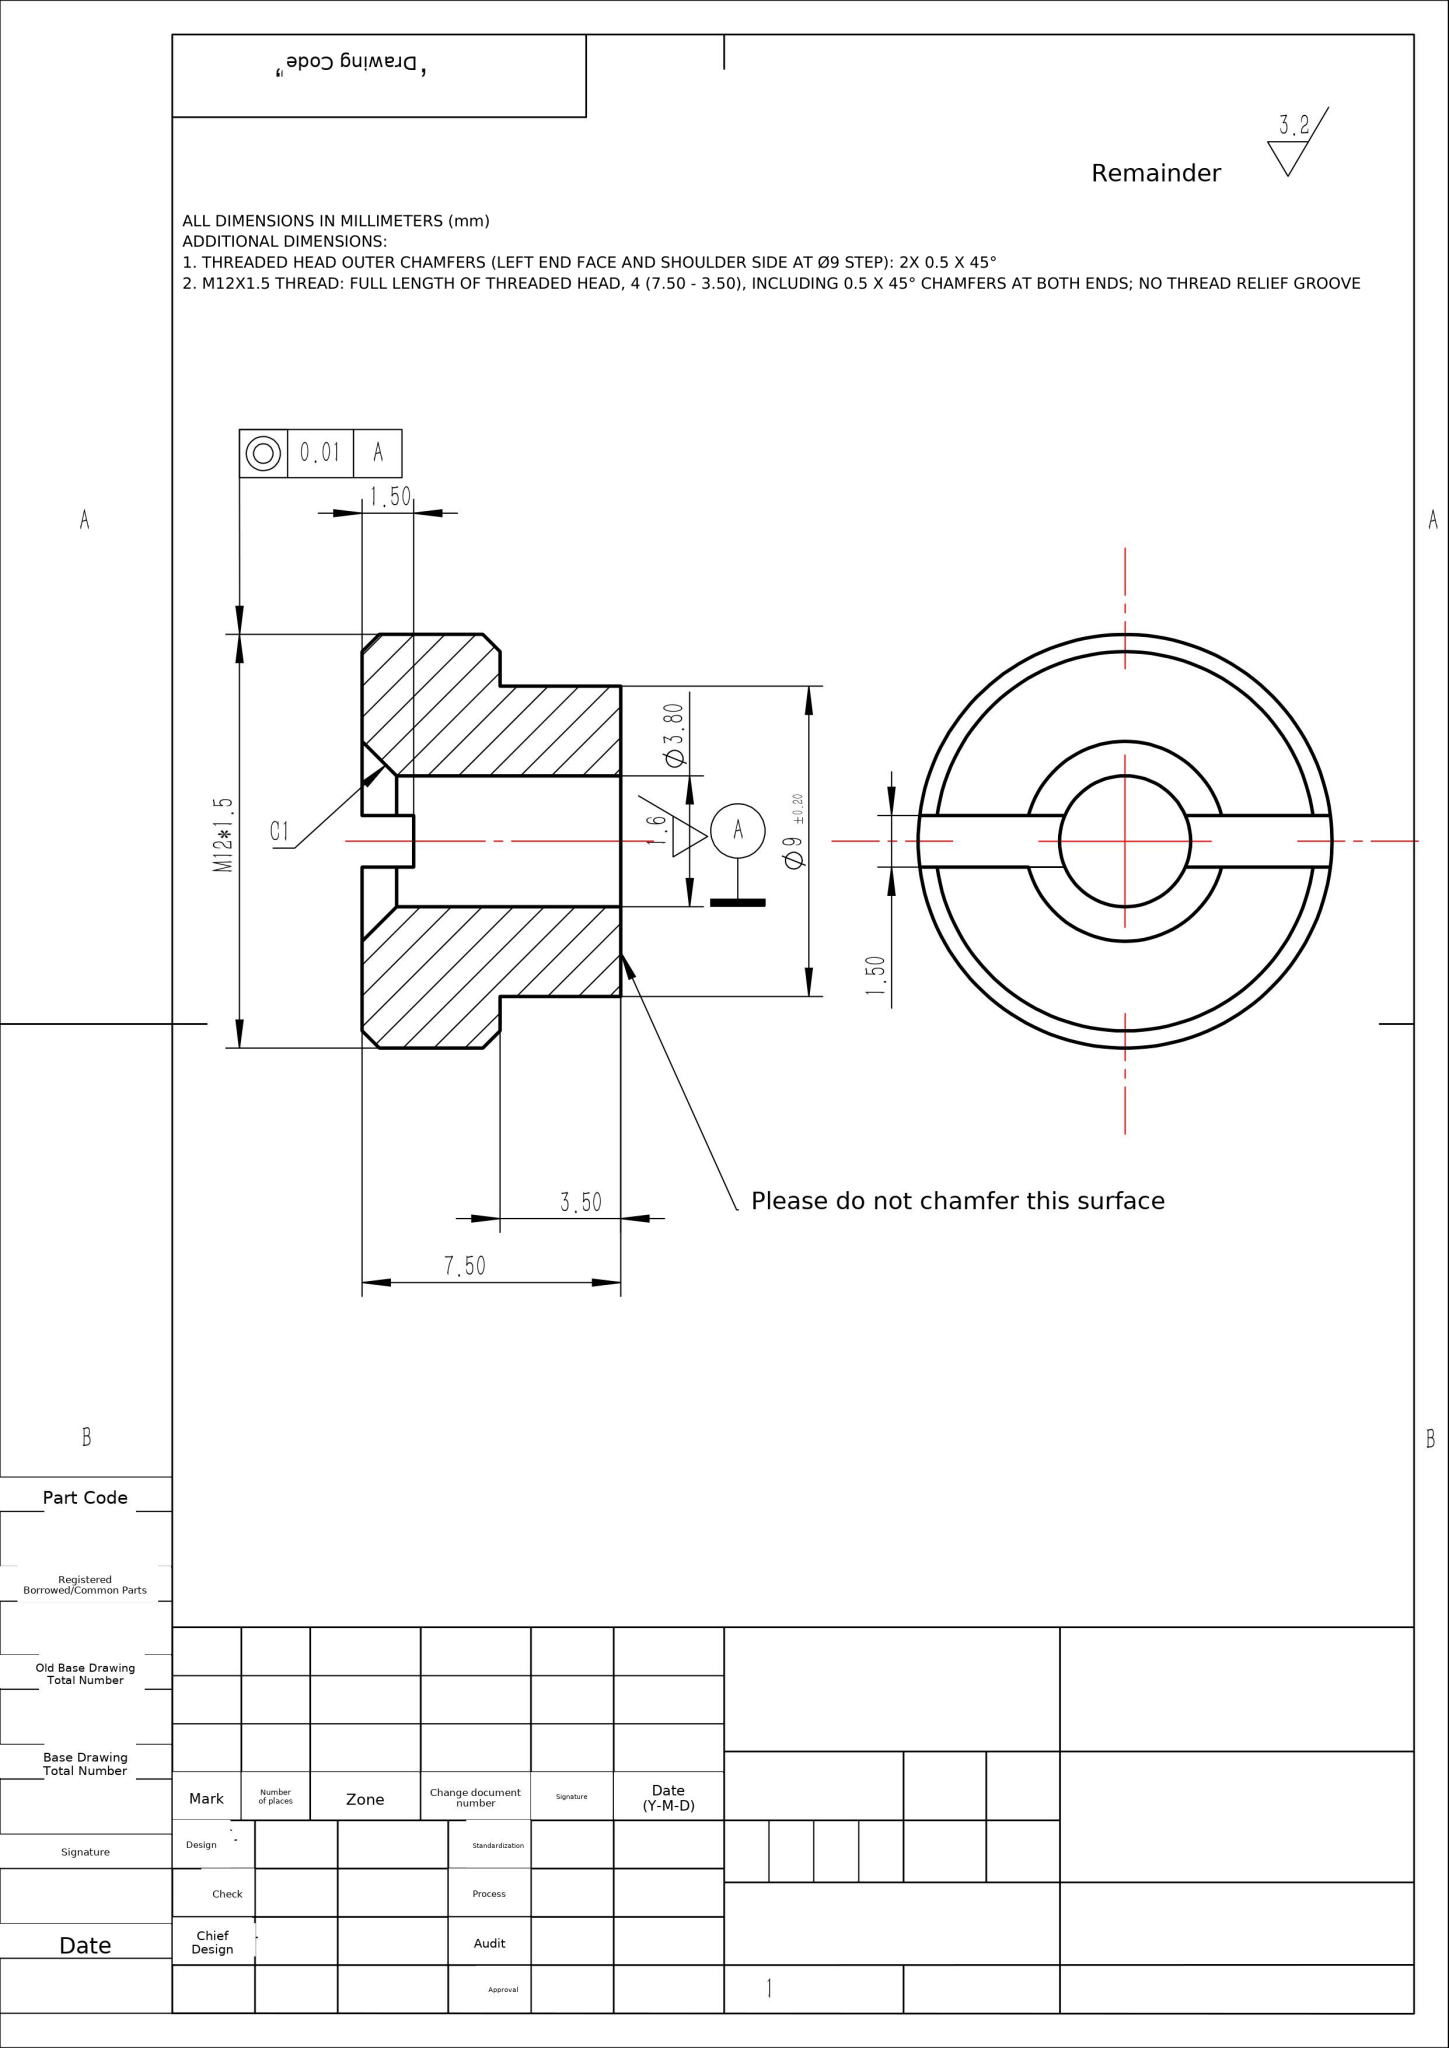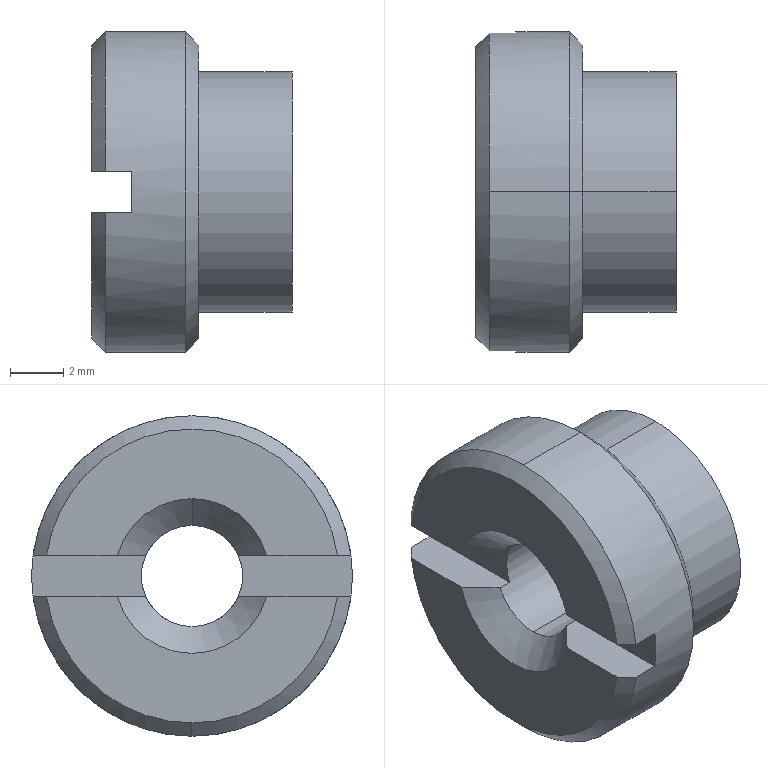Part | NX | mm | 1 solid | 24 faces | box 7.5 x 12 x 12 mm | volume 557 mm3 | plane 10 | cone 8 | cylinder 6 | commonest cylinder face diameters 3.8 x2 9 x2 12 x2
STEP:
#1=COLOUR_RGB('',0.6471,0.5176,0.);
#2=FILL_AREA_STYLE_COLOUR('',#1);
#3=FILL_AREA_STYLE('',(#2));
#4=SURFACE_STYLE_FILL_AREA(#3);
#5=SURFACE_SIDE_STYLE('',(#4));
#6=SURFACE_STYLE_USAGE(.BOTH.,#5);
#7=PRESENTATION_STYLE_ASSIGNMENT((#6));
#8=CARTESIAN_POINT('',(1.,-1.746,0.75));
#9=VERTEX_POINT('',#8);
#10=CARTESIAN_POINT('',(1.,-0.,1.9));
#11=VERTEX_POINT('',#10);
#12=CARTESIAN_POINT('',(1.,0.,0.));
#13=DIRECTION('',(-1.,0.,0.));
#14=DIRECTION('',(0.,0.,-1.));
#15=AXIS2_PLACEMENT_3D('',#12,#13,#14);
#16=CIRCLE('',#15,1.9);
#17=EDGE_CURVE('',#9,#11,#16,.T.);
#18=ORIENTED_EDGE('',*,*,#17,.T.);
#19=CARTESIAN_POINT('',(7.5,0.,1.9));
#20=VERTEX_POINT('',#19);
#21=CARTESIAN_POINT('',(0.,0.,1.9));
#22=DIRECTION('',(1.,0.,0.));
#23=VECTOR('',#22,1000.);
#24=LINE('',#21,#23);
#25=EDGE_CURVE('',#11,#20,#24,.T.);
#26=ORIENTED_EDGE('',*,*,#25,.T.);
#27=CARTESIAN_POINT('',(7.5,0.,-1.9));
#28=VERTEX_POINT('',#27);
#29=CARTESIAN_POINT('',(7.5,0.,0.));
#30=DIRECTION('',(1.,0.,0.));
#31=DIRECTION('',(0.,0.,-1.));
#32=AXIS2_PLACEMENT_3D('',#29,#30,#31);
#33=CIRCLE('',#32,1.9);
#34=EDGE_CURVE('',#20,#28,#33,.T.);
#35=ORIENTED_EDGE('',*,*,#34,.T.);
#36=CARTESIAN_POINT('',(1.,0.,-1.9));
#37=VERTEX_POINT('',#36);
#38=CARTESIAN_POINT('',(0.,0.,-1.9));
#39=DIRECTION('',(1.,0.,0.));
#40=VECTOR('',#39,1000.);
#41=LINE('',#38,#40);
#42=EDGE_CURVE('',#37,#28,#41,.T.);
#43=ORIENTED_EDGE('',*,*,#42,.F.);
#44=CARTESIAN_POINT('',(1.,-1.746,-0.75));
#45=VERTEX_POINT('',#44);
#46=CARTESIAN_POINT('',(1.,0.,0.));
#47=DIRECTION('',(-1.,0.,0.));
#48=DIRECTION('',(0.,0.,-1.));
#49=AXIS2_PLACEMENT_3D('',#46,#47,#48);
#50=CIRCLE('',#49,1.9);
#51=EDGE_CURVE('',#37,#45,#50,.T.);
#52=ORIENTED_EDGE('',*,*,#51,.T.);
#53=CARTESIAN_POINT('',(1.5,-1.746,-0.75));
#54=VERTEX_POINT('',#53);
#55=CARTESIAN_POINT('',(0.,-1.746,-0.75));
#56=DIRECTION('',(1.,0.,0.));
#57=VECTOR('',#56,1000.);
#58=LINE('',#55,#57);
#59=EDGE_CURVE('',#45,#54,#58,.T.);
#60=ORIENTED_EDGE('',*,*,#59,.T.);
#61=CARTESIAN_POINT('',(1.5,-1.746,0.75));
#62=VERTEX_POINT('',#61);
#63=CARTESIAN_POINT('',(1.5,0.,0.));
#64=DIRECTION('',(-1.,0.,0.));
#65=DIRECTION('',(0.,0.,-1.));
#66=AXIS2_PLACEMENT_3D('',#63,#64,#65);
#67=CIRCLE('',#66,1.9);
#68=EDGE_CURVE('',#54,#62,#67,.T.);
#69=ORIENTED_EDGE('',*,*,#68,.T.);
#70=CARTESIAN_POINT('',(0.,-1.746,0.75));
#71=DIRECTION('',(-1.,0.,0.));
#72=VECTOR('',#71,1000.);
#73=LINE('',#70,#72);
#74=EDGE_CURVE('',#62,#9,#73,.T.);
#75=ORIENTED_EDGE('',*,*,#74,.T.);
#76=EDGE_LOOP('',(#18,#26,#35,#43,#52,#60,#69,#75));
#77=FACE_OUTER_BOUND('',#76,.T.);
#78=CARTESIAN_POINT('',(0.,0.,0.));
#79=DIRECTION('',(1.,0.,0.));
#80=DIRECTION('',(0.,0.,-1.));
#81=AXIS2_PLACEMENT_3D('',#78,#79,#80);
#82=CYLINDRICAL_SURFACE('',#81,1.9);
#83=ADVANCED_FACE('',(#77),#82,.F.);
#84=CARTESIAN_POINT('',(4.,0.,-5.5));
#85=VERTEX_POINT('',#84);
#86=CARTESIAN_POINT('',(4.,-0.,5.5));
#87=VERTEX_POINT('',#86);
#88=CARTESIAN_POINT('',(4.,0.,0.));
#89=DIRECTION('',(1.,0.,0.));
#90=DIRECTION('',(0.,0.,-1.));
#91=AXIS2_PLACEMENT_3D('',#88,#89,#90);
#92=CIRCLE('',#91,5.5);
#93=EDGE_CURVE('',#85,#87,#92,.T.);
#94=ORIENTED_EDGE('',*,*,#93,.F.);
#95=CARTESIAN_POINT('',(3.5,0.,-6.));
#96=VERTEX_POINT('',#95);
#97=CARTESIAN_POINT('',(4.,0.,-5.5));
#98=DIRECTION('',(-0.7071,0.,-0.7071));
#99=VECTOR('',#98,1000.);
#100=LINE('',#97,#99);
#101=EDGE_CURVE('',#85,#96,#100,.T.);
#102=ORIENTED_EDGE('',*,*,#101,.T.);
#103=CARTESIAN_POINT('',(3.5,-0.,6.));
#104=VERTEX_POINT('',#103);
#105=CARTESIAN_POINT('',(3.5,0.,0.));
#106=DIRECTION('',(-1.,0.,0.));
#107=DIRECTION('',(0.,0.,-1.));
#108=AXIS2_PLACEMENT_3D('',#105,#106,#107);
#109=CIRCLE('',#108,6.);
#110=EDGE_CURVE('',#104,#96,#109,.T.);
#111=ORIENTED_EDGE('',*,*,#110,.F.);
#112=CARTESIAN_POINT('',(4.,-0.,5.5));
#113=DIRECTION('',(-0.7071,-0.,0.7071));
#114=VECTOR('',#113,1000.);
#115=LINE('',#112,#114);
#116=EDGE_CURVE('',#87,#104,#115,.T.);
#117=ORIENTED_EDGE('',*,*,#116,.F.);
#118=EDGE_LOOP('',(#94,#102,#111,#117));
#119=FACE_OUTER_BOUND('',#118,.T.);
#120=CARTESIAN_POINT('',(4.,0.,0.));
#121=DIRECTION('',(-1.,0.,0.));
#122=DIRECTION('',(0.,-0.,1.));
#123=AXIS2_PLACEMENT_3D('',#120,#121,#122);
#124=CONICAL_SURFACE('',#123,5.5,0.7854);
#125=ADVANCED_FACE('',(#119),#124,.T.);
#126=CARTESIAN_POINT('',(0.,0.,-5.5));
#127=VERTEX_POINT('',#126);
#128=CARTESIAN_POINT('',(0.,-5.449,-0.75));
#129=VERTEX_POINT('',#128);
#130=CARTESIAN_POINT('',(0.,0.,0.));
#131=DIRECTION('',(-1.,0.,0.));
#132=DIRECTION('',(0.,0.,-1.));
#133=AXIS2_PLACEMENT_3D('',#130,#131,#132);
#134=CIRCLE('',#133,5.5);
#135=EDGE_CURVE('',#127,#129,#134,.T.);
#136=ORIENTED_EDGE('',*,*,#135,.F.);
#137=CARTESIAN_POINT('',(0.5,0.,-6.));
#138=VERTEX_POINT('',#137);
#139=CARTESIAN_POINT('',(0.5,0.,-6.));
#140=DIRECTION('',(0.7071,0.,-0.7071));
#141=VECTOR('',#140,1000.);
#142=LINE('',#139,#141);
#143=EDGE_CURVE('',#127,#138,#142,.T.);
#144=ORIENTED_EDGE('',*,*,#143,.T.);
#145=CARTESIAN_POINT('',(0.5,-5.953,-0.75));
#146=VERTEX_POINT('',#145);
#147=CARTESIAN_POINT('',(0.5,0.,0.));
#148=DIRECTION('',(1.,0.,0.));
#149=DIRECTION('',(0.,0.,-1.));
#150=AXIS2_PLACEMENT_3D('',#147,#148,#149);
#151=CIRCLE('',#150,6.);
#152=EDGE_CURVE('',#146,#138,#151,.T.);
#153=ORIENTED_EDGE('',*,*,#152,.F.);
#154=CARTESIAN_POINT('',(0.,-5.449,-0.75));
#155=CARTESIAN_POINT('',(0.1666,-5.617,-0.75));
#156=CARTESIAN_POINT('',(0.3333,-5.785,-0.75));
#157=CARTESIAN_POINT('',(0.5,-5.953,-0.75));
#158=B_SPLINE_CURVE_WITH_KNOTS('',3,(#154,#155,#156,#157),.UNSPECIFIED.,.F.,.F.,(4,4),(0.02551,0.02623),.UNSPECIFIED.);
#159=EDGE_CURVE('',#129,#146,#158,.T.);
#160=ORIENTED_EDGE('',*,*,#159,.F.);
#161=EDGE_LOOP('',(#136,#144,#153,#160));
#162=FACE_OUTER_BOUND('',#161,.T.);
#163=CARTESIAN_POINT('',(0.5,0.,0.));
#164=DIRECTION('',(1.,0.,0.));
#165=DIRECTION('',(0.,0.,-1.));
#166=AXIS2_PLACEMENT_3D('',#163,#164,#165);
#167=CONICAL_SURFACE('',#166,6.,0.7854);
#168=ADVANCED_FACE('',(#162),#167,.T.);
#169=CARTESIAN_POINT('',(7.5,0.,-4.5));
#170=VERTEX_POINT('',#169);
#171=CARTESIAN_POINT('',(7.5,-0.,4.5));
#172=VERTEX_POINT('',#171);
#173=CARTESIAN_POINT('',(7.5,0.,0.));
#174=DIRECTION('',(1.,0.,0.));
#175=DIRECTION('',(0.,0.,-1.));
#176=AXIS2_PLACEMENT_3D('',#173,#174,#175);
#177=CIRCLE('',#176,4.5);
#178=EDGE_CURVE('',#170,#172,#177,.T.);
#179=ORIENTED_EDGE('',*,*,#178,.F.);
#180=CARTESIAN_POINT('',(4.,0.,-4.5));
#181=VERTEX_POINT('',#180);
#182=CARTESIAN_POINT('',(7.5,0.,-4.5));
#183=DIRECTION('',(-1.,0.,0.));
#184=VECTOR('',#183,1000.);
#185=LINE('',#182,#184);
#186=EDGE_CURVE('',#170,#181,#185,.T.);
#187=ORIENTED_EDGE('',*,*,#186,.T.);
#188=CARTESIAN_POINT('',(4.,-0.,4.5));
#189=VERTEX_POINT('',#188);
#190=CARTESIAN_POINT('',(4.,0.,0.));
#191=DIRECTION('',(1.,0.,0.));
#192=DIRECTION('',(0.,0.,-1.));
#193=AXIS2_PLACEMENT_3D('',#190,#191,#192);
#194=CIRCLE('',#193,4.5);
#195=EDGE_CURVE('',#181,#189,#194,.T.);
#196=ORIENTED_EDGE('',*,*,#195,.T.);
#197=CARTESIAN_POINT('',(7.5,-0.,4.5));
#198=DIRECTION('',(-1.,0.,0.));
#199=VECTOR('',#198,1000.);
#200=LINE('',#197,#199);
#201=EDGE_CURVE('',#172,#189,#200,.T.);
#202=ORIENTED_EDGE('',*,*,#201,.F.);
#203=EDGE_LOOP('',(#179,#187,#196,#202));
#204=FACE_OUTER_BOUND('',#203,.T.);
#205=CARTESIAN_POINT('',(7.5,0.,0.));
#206=DIRECTION('',(-1.,0.,0.));
#207=DIRECTION('',(0.,-0.,1.));
#208=AXIS2_PLACEMENT_3D('',#205,#206,#207);
#209=CYLINDRICAL_SURFACE('',#208,4.5);
#210=ADVANCED_FACE('',(#204),#209,.T.);
#211=ORIENTED_EDGE('',*,*,#110,.T.);
#212=CARTESIAN_POINT('',(4.,0.,-6.));
#213=DIRECTION('',(-1.,0.,0.));
#214=VECTOR('',#213,1000.);
#215=LINE('',#212,#214);
#216=EDGE_CURVE('',#96,#138,#215,.T.);
#217=ORIENTED_EDGE('',*,*,#216,.T.);
#218=CARTESIAN_POINT('',(0.5,5.953,-0.75));
#219=VERTEX_POINT('',#218);
#220=CARTESIAN_POINT('',(0.5,0.,0.));
#221=DIRECTION('',(1.,0.,0.));
#222=DIRECTION('',(0.,0.,-1.));
#223=AXIS2_PLACEMENT_3D('',#220,#221,#222);
#224=CIRCLE('',#223,6.);
#225=EDGE_CURVE('',#138,#219,#224,.T.);
#226=ORIENTED_EDGE('',*,*,#225,.T.);
#227=CARTESIAN_POINT('',(1.5,5.953,-0.75));
#228=VERTEX_POINT('',#227);
#229=CARTESIAN_POINT('',(4.,5.953,-0.75));
#230=DIRECTION('',(1.,0.,0.));
#231=VECTOR('',#230,1000.);
#232=LINE('',#229,#231);
#233=EDGE_CURVE('',#219,#228,#232,.T.);
#234=ORIENTED_EDGE('',*,*,#233,.T.);
#235=CARTESIAN_POINT('',(1.5,5.953,0.75));
#236=VERTEX_POINT('',#235);
#237=CARTESIAN_POINT('',(1.5,0.,0.));
#238=DIRECTION('',(1.,0.,0.));
#239=DIRECTION('',(0.,0.,-1.));
#240=AXIS2_PLACEMENT_3D('',#237,#238,#239);
#241=CIRCLE('',#240,6.);
#242=EDGE_CURVE('',#228,#236,#241,.T.);
#243=ORIENTED_EDGE('',*,*,#242,.T.);
#244=CARTESIAN_POINT('',(0.5,5.953,0.75));
#245=VERTEX_POINT('',#244);
#246=CARTESIAN_POINT('',(4.,5.953,0.75));
#247=DIRECTION('',(-1.,0.,0.));
#248=VECTOR('',#247,1000.);
#249=LINE('',#246,#248);
#250=EDGE_CURVE('',#236,#245,#249,.T.);
#251=ORIENTED_EDGE('',*,*,#250,.T.);
#252=CARTESIAN_POINT('',(0.5,-0.,6.));
#253=VERTEX_POINT('',#252);
#254=CARTESIAN_POINT('',(0.5,0.,0.));
#255=DIRECTION('',(1.,0.,0.));
#256=DIRECTION('',(0.,0.,-1.));
#257=AXIS2_PLACEMENT_3D('',#254,#255,#256);
#258=CIRCLE('',#257,6.);
#259=EDGE_CURVE('',#245,#253,#258,.T.);
#260=ORIENTED_EDGE('',*,*,#259,.T.);
#261=CARTESIAN_POINT('',(4.,-0.,6.));
#262=DIRECTION('',(-1.,0.,0.));
#263=VECTOR('',#262,1000.);
#264=LINE('',#261,#263);
#265=EDGE_CURVE('',#104,#253,#264,.T.);
#266=ORIENTED_EDGE('',*,*,#265,.F.);
#267=EDGE_LOOP('',(#211,#217,#226,#234,#243,#251,#260,#266));
#268=FACE_OUTER_BOUND('',#267,.T.);
#269=CARTESIAN_POINT('',(4.,0.,0.));
#270=DIRECTION('',(-1.,0.,0.));
#271=DIRECTION('',(0.,-0.,1.));
#272=AXIS2_PLACEMENT_3D('',#269,#270,#271);
#273=CYLINDRICAL_SURFACE('',#272,6.);
#274=ADVANCED_FACE('',(#268),#273,.T.);
#275=CARTESIAN_POINT('',(1.,1.746,0.75));
#276=VERTEX_POINT('',#275);
#277=CARTESIAN_POINT('',(1.,0.,0.));
#278=DIRECTION('',(-1.,0.,0.));
#279=DIRECTION('',(0.,0.,-1.));
#280=AXIS2_PLACEMENT_3D('',#277,#278,#279);
#281=CIRCLE('',#280,1.9);
#282=EDGE_CURVE('',#11,#276,#281,.T.);
#283=ORIENTED_EDGE('',*,*,#282,.F.);
#284=CARTESIAN_POINT('',(0.,-0.,2.9));
#285=VERTEX_POINT('',#284);
#286=CARTESIAN_POINT('',(0.,-0.,2.9));
#287=DIRECTION('',(-0.7071,-0.,0.7071));
#288=VECTOR('',#287,1000.);
#289=LINE('',#286,#288);
#290=EDGE_CURVE('',#11,#285,#289,.T.);
#291=ORIENTED_EDGE('',*,*,#290,.T.);
#292=CARTESIAN_POINT('',(0.,2.801,0.75));
#293=VERTEX_POINT('',#292);
#294=CARTESIAN_POINT('',(0.,0.,0.));
#295=DIRECTION('',(1.,0.,0.));
#296=DIRECTION('',(0.,0.,-1.));
#297=AXIS2_PLACEMENT_3D('',#294,#295,#296);
#298=CIRCLE('',#297,2.9);
#299=EDGE_CURVE('',#293,#285,#298,.T.);
#300=ORIENTED_EDGE('',*,*,#299,.F.);
#301=CARTESIAN_POINT('',(1.,1.746,0.75));
#302=CARTESIAN_POINT('',(0.6721,2.103,0.75));
#303=CARTESIAN_POINT('',(0.3368,2.453,0.75));
#304=CARTESIAN_POINT('',(0.,2.801,0.75));
#305=B_SPLINE_CURVE_WITH_KNOTS('',3,(#301,#302,#303,#304),.UNSPECIFIED.,.F.,.F.,(4,4),(0.0107,0.01214),.UNSPECIFIED.);
#306=EDGE_CURVE('',#276,#293,#305,.T.);
#307=ORIENTED_EDGE('',*,*,#306,.F.);
#308=EDGE_LOOP('',(#283,#291,#300,#307));
#309=FACE_OUTER_BOUND('',#308,.T.);
#310=CARTESIAN_POINT('',(0.,0.,0.));
#311=DIRECTION('',(-1.,0.,0.));
#312=DIRECTION('',(0.,-0.,1.));
#313=AXIS2_PLACEMENT_3D('',#310,#311,#312);
#314=CONICAL_SURFACE('',#313,2.9,0.7854);
#315=ADVANCED_FACE('',(#309),#314,.F.);
#316=CARTESIAN_POINT('',(0.,-5.449,0.75));
#317=VERTEX_POINT('',#316);
#318=CARTESIAN_POINT('',(0.,5.449,0.75));
#319=VERTEX_POINT('',#318);
#320=CARTESIAN_POINT('',(0.,0.,0.));
#321=DIRECTION('',(-1.,0.,0.));
#322=DIRECTION('',(0.,0.,-1.));
#323=AXIS2_PLACEMENT_3D('',#320,#321,#322);
#324=CIRCLE('',#323,5.5);
#325=EDGE_CURVE('',#317,#319,#324,.T.);
#326=ORIENTED_EDGE('',*,*,#325,.T.);
#327=CARTESIAN_POINT('',(0.,0.,0.75));
#328=DIRECTION('',(0.,-1.,-0.));
#329=VECTOR('',#328,1000.);
#330=LINE('',#327,#329);
#331=EDGE_CURVE('',#319,#293,#330,.T.);
#332=ORIENTED_EDGE('',*,*,#331,.T.);
#333=ORIENTED_EDGE('',*,*,#299,.T.);
#334=CARTESIAN_POINT('',(0.,-2.801,0.75));
#335=VERTEX_POINT('',#334);
#336=CARTESIAN_POINT('',(0.,0.,0.));
#337=DIRECTION('',(1.,0.,0.));
#338=DIRECTION('',(0.,0.,-1.));
#339=AXIS2_PLACEMENT_3D('',#336,#337,#338);
#340=CIRCLE('',#339,2.9);
#341=EDGE_CURVE('',#285,#335,#340,.T.);
#342=ORIENTED_EDGE('',*,*,#341,.T.);
#343=CARTESIAN_POINT('',(0.,0.,0.75));
#344=DIRECTION('',(0.,-1.,-0.));
#345=VECTOR('',#344,1000.);
#346=LINE('',#343,#345);
#347=EDGE_CURVE('',#335,#317,#346,.T.);
#348=ORIENTED_EDGE('',*,*,#347,.T.);
#349=EDGE_LOOP('',(#326,#332,#333,#342,#348));
#350=FACE_OUTER_BOUND('',#349,.T.);
#351=CARTESIAN_POINT('',(0.,0.,0.));
#352=DIRECTION('',(1.,0.,0.));
#353=DIRECTION('',(0.,0.,-1.));
#354=AXIS2_PLACEMENT_3D('',#351,#352,#353);
#355=PLANE('',#354);
#356=ADVANCED_FACE('',(#350),#355,.F.);
#357=CARTESIAN_POINT('',(0.5,-5.953,0.75));
#358=VERTEX_POINT('',#357);
#359=CARTESIAN_POINT('',(0.5,-5.953,0.75));
#360=CARTESIAN_POINT('',(0.3333,-5.785,0.75));
#361=CARTESIAN_POINT('',(0.1666,-5.617,0.75));
#362=CARTESIAN_POINT('',(0.,-5.449,0.75));
#363=B_SPLINE_CURVE_WITH_KNOTS('',3,(#359,#360,#361,#362),.UNSPECIFIED.,.F.,.F.,(4,4),(0.01021,0.01092),.UNSPECIFIED.);
#364=EDGE_CURVE('',#358,#317,#363,.T.);
#365=ORIENTED_EDGE('',*,*,#364,.F.);
#366=CARTESIAN_POINT('',(0.5,0.,0.));
#367=DIRECTION('',(1.,0.,0.));
#368=DIRECTION('',(0.,0.,-1.));
#369=AXIS2_PLACEMENT_3D('',#366,#367,#368);
#370=CIRCLE('',#369,6.);
#371=EDGE_CURVE('',#253,#358,#370,.T.);
#372=ORIENTED_EDGE('',*,*,#371,.F.);
#373=ORIENTED_EDGE('',*,*,#259,.F.);
#374=CARTESIAN_POINT('',(0.,5.449,0.75));
#375=CARTESIAN_POINT('',(0.1666,5.617,0.75));
#376=CARTESIAN_POINT('',(0.3333,5.785,0.75));
#377=CARTESIAN_POINT('',(0.5,5.953,0.75));
#378=B_SPLINE_CURVE_WITH_KNOTS('',3,(#374,#375,#376,#377),.UNSPECIFIED.,.F.,.F.,(4,4),(0.02551,0.02623),.UNSPECIFIED.);
#379=EDGE_CURVE('',#319,#245,#378,.T.);
#380=ORIENTED_EDGE('',*,*,#379,.F.);
#381=ORIENTED_EDGE('',*,*,#325,.F.);
#382=EDGE_LOOP('',(#365,#372,#373,#380,#381));
#383=FACE_OUTER_BOUND('',#382,.T.);
#384=CARTESIAN_POINT('',(0.5,0.,0.));
#385=DIRECTION('',(1.,0.,0.));
#386=DIRECTION('',(0.,0.,-1.));
#387=AXIS2_PLACEMENT_3D('',#384,#385,#386);
#388=CONICAL_SURFACE('',#387,6.,0.7854);
#389=ADVANCED_FACE('',(#383),#388,.T.);
#390=ORIENTED_EDGE('',*,*,#290,.F.);
#391=ORIENTED_EDGE('',*,*,#17,.F.);
#392=CARTESIAN_POINT('',(0.,-2.801,0.75));
#393=CARTESIAN_POINT('',(0.3367,-2.453,0.75));
#394=CARTESIAN_POINT('',(0.672,-2.103,0.75));
#395=CARTESIAN_POINT('',(1.,-1.746,0.75));
#396=B_SPLINE_CURVE_WITH_KNOTS('',3,(#392,#393,#394,#395),.UNSPECIFIED.,.F.,.F.,(4,4),(0.005033,0.006487),.UNSPECIFIED.);
#397=EDGE_CURVE('',#335,#9,#396,.T.);
#398=ORIENTED_EDGE('',*,*,#397,.F.);
#399=ORIENTED_EDGE('',*,*,#341,.F.);
#400=EDGE_LOOP('',(#390,#391,#398,#399));
#401=FACE_OUTER_BOUND('',#400,.T.);
#402=CARTESIAN_POINT('',(0.,0.,0.));
#403=DIRECTION('',(-1.,0.,0.));
#404=DIRECTION('',(0.,-0.,1.));
#405=AXIS2_PLACEMENT_3D('',#402,#403,#404);
#406=CONICAL_SURFACE('',#405,2.9,0.7854);
#407=ADVANCED_FACE('',(#401),#406,.F.);
#408=CARTESIAN_POINT('',(4.,0.,0.));
#409=DIRECTION('',(1.,0.,0.));
#410=DIRECTION('',(0.,0.,-1.));
#411=AXIS2_PLACEMENT_3D('',#408,#409,#410);
#412=CIRCLE('',#411,5.5);
#413=EDGE_CURVE('',#87,#85,#412,.T.);
#414=ORIENTED_EDGE('',*,*,#413,.T.);
#415=ORIENTED_EDGE('',*,*,#93,.T.);
#416=EDGE_LOOP('',(#414,#415));
#417=FACE_OUTER_BOUND('',#416,.T.);
#418=CARTESIAN_POINT('',(4.,0.,0.));
#419=DIRECTION('',(1.,0.,0.));
#420=DIRECTION('',(0.,0.,-1.));
#421=AXIS2_PLACEMENT_3D('',#418,#419,#420);
#422=CIRCLE('',#421,4.5);
#423=EDGE_CURVE('',#189,#181,#422,.T.);
#424=ORIENTED_EDGE('',*,*,#423,.F.);
#425=ORIENTED_EDGE('',*,*,#195,.F.);
#426=EDGE_LOOP('',(#424,#425));
#427=FACE_BOUND('',#426,.T.);
#428=CARTESIAN_POINT('',(4.,0.,0.));
#429=DIRECTION('',(1.,0.,0.));
#430=DIRECTION('',(0.,0.,-1.));
#431=AXIS2_PLACEMENT_3D('',#428,#429,#430);
#432=PLANE('',#431);
#433=ADVANCED_FACE('',(#417,#427),#432,.T.);
#434=ORIENTED_EDGE('',*,*,#216,.F.);
#435=CARTESIAN_POINT('',(3.5,0.,0.));
#436=DIRECTION('',(-1.,0.,0.));
#437=DIRECTION('',(0.,0.,-1.));
#438=AXIS2_PLACEMENT_3D('',#435,#436,#437);
#439=CIRCLE('',#438,6.);
#440=EDGE_CURVE('',#96,#104,#439,.T.);
#441=ORIENTED_EDGE('',*,*,#440,.T.);
#442=ORIENTED_EDGE('',*,*,#265,.T.);
#443=ORIENTED_EDGE('',*,*,#371,.T.);
#444=CARTESIAN_POINT('',(1.5,-5.953,0.75));
#445=VERTEX_POINT('',#444);
#446=CARTESIAN_POINT('',(4.,-5.953,0.75));
#447=DIRECTION('',(1.,0.,0.));
#448=VECTOR('',#447,1000.);
#449=LINE('',#446,#448);
#450=EDGE_CURVE('',#358,#445,#449,.T.);
#451=ORIENTED_EDGE('',*,*,#450,.T.);
#452=CARTESIAN_POINT('',(1.5,-5.953,-0.75));
#453=VERTEX_POINT('',#452);
#454=CARTESIAN_POINT('',(1.5,0.,0.));
#455=DIRECTION('',(1.,0.,0.));
#456=DIRECTION('',(0.,0.,-1.));
#457=AXIS2_PLACEMENT_3D('',#454,#455,#456);
#458=CIRCLE('',#457,6.);
#459=EDGE_CURVE('',#445,#453,#458,.T.);
#460=ORIENTED_EDGE('',*,*,#459,.T.);
#461=CARTESIAN_POINT('',(4.,-5.953,-0.75));
#462=DIRECTION('',(-1.,0.,0.));
#463=VECTOR('',#462,1000.);
#464=LINE('',#461,#463);
#465=EDGE_CURVE('',#453,#146,#464,.T.);
#466=ORIENTED_EDGE('',*,*,#465,.T.);
#467=ORIENTED_EDGE('',*,*,#152,.T.);
#468=EDGE_LOOP('',(#434,#441,#442,#443,#451,#460,#466,#467));
#469=FACE_OUTER_BOUND('',#468,.T.);
#470=CARTESIAN_POINT('',(4.,0.,0.));
#471=DIRECTION('',(-1.,0.,0.));
#472=DIRECTION('',(0.,-0.,1.));
#473=AXIS2_PLACEMENT_3D('',#470,#471,#472);
#474=CYLINDRICAL_SURFACE('',#473,6.);
#475=ADVANCED_FACE('',(#469),#474,.T.);
#476=CARTESIAN_POINT('',(0.,5.449,-0.75));
#477=VERTEX_POINT('',#476);
#478=CARTESIAN_POINT('',(0.,0.,0.));
#479=DIRECTION('',(-1.,0.,0.));
#480=DIRECTION('',(0.,-0.,-1.));
#481=AXIS2_PLACEMENT_3D('',#478,#479,#480);
#482=CIRCLE('',#481,5.5);
#483=EDGE_CURVE('',#477,#127,#482,.T.);
#484=ORIENTED_EDGE('',*,*,#483,.T.);
#485=ORIENTED_EDGE('',*,*,#135,.T.);
#486=CARTESIAN_POINT('',(0.,-2.801,-0.75));
#487=VERTEX_POINT('',#486);
#488=CARTESIAN_POINT('',(0.,0.,-0.75));
#489=DIRECTION('',(0.,1.,0.));
#490=VECTOR('',#489,1000.);
#491=LINE('',#488,#490);
#492=EDGE_CURVE('',#129,#487,#491,.T.);
#493=ORIENTED_EDGE('',*,*,#492,.T.);
#494=CARTESIAN_POINT('',(0.,2.801,-0.75));
#495=VERTEX_POINT('',#494);
#496=CARTESIAN_POINT('',(0.,0.,0.));
#497=DIRECTION('',(1.,0.,0.));
#498=DIRECTION('',(0.,0.,-1.));
#499=AXIS2_PLACEMENT_3D('',#496,#497,#498);
#500=CIRCLE('',#499,2.9);
#501=EDGE_CURVE('',#487,#495,#500,.T.);
#502=ORIENTED_EDGE('',*,*,#501,.T.);
#503=CARTESIAN_POINT('',(0.,0.,-0.75));
#504=DIRECTION('',(0.,1.,0.));
#505=VECTOR('',#504,1000.);
#506=LINE('',#503,#505);
#507=EDGE_CURVE('',#495,#477,#506,.T.);
#508=ORIENTED_EDGE('',*,*,#507,.T.);
#509=EDGE_LOOP('',(#484,#485,#493,#502,#508));
#510=FACE_OUTER_BOUND('',#509,.T.);
#511=CARTESIAN_POINT('',(0.,0.,0.));
#512=DIRECTION('',(1.,0.,0.));
#513=DIRECTION('',(0.,0.,-1.));
#514=AXIS2_PLACEMENT_3D('',#511,#512,#513);
#515=PLANE('',#514);
#516=ADVANCED_FACE('',(#510),#515,.F.);
#517=ORIENTED_EDGE('',*,*,#186,.F.);
#518=CARTESIAN_POINT('',(7.5,0.,0.));
#519=DIRECTION('',(1.,0.,0.));
#520=DIRECTION('',(0.,0.,-1.));
#521=AXIS2_PLACEMENT_3D('',#518,#519,#520);
#522=CIRCLE('',#521,4.5);
#523=EDGE_CURVE('',#172,#170,#522,.T.);
#524=ORIENTED_EDGE('',*,*,#523,.F.);
#525=ORIENTED_EDGE('',*,*,#201,.T.);
#526=ORIENTED_EDGE('',*,*,#423,.T.);
#527=EDGE_LOOP('',(#517,#524,#525,#526));
#528=FACE_OUTER_BOUND('',#527,.T.);
#529=CARTESIAN_POINT('',(7.5,0.,0.));
#530=DIRECTION('',(-1.,0.,0.));
#531=DIRECTION('',(0.,-0.,1.));
#532=AXIS2_PLACEMENT_3D('',#529,#530,#531);
#533=CYLINDRICAL_SURFACE('',#532,4.5);
#534=ADVANCED_FACE('',(#528),#533,.T.);
#535=CARTESIAN_POINT('',(7.5,0.,0.));
#536=DIRECTION('',(1.,0.,0.));
#537=DIRECTION('',(0.,0.,-1.));
#538=AXIS2_PLACEMENT_3D('',#535,#536,#537);
#539=CIRCLE('',#538,1.9);
#540=EDGE_CURVE('',#28,#20,#539,.T.);
#541=ORIENTED_EDGE('',*,*,#540,.F.);
#542=ORIENTED_EDGE('',*,*,#34,.F.);
#543=EDGE_LOOP('',(#541,#542));
#544=FACE_BOUND('',#543,.T.);
#545=ORIENTED_EDGE('',*,*,#523,.T.);
#546=ORIENTED_EDGE('',*,*,#178,.T.);
#547=EDGE_LOOP('',(#545,#546));
#548=FACE_OUTER_BOUND('',#547,.T.);
#549=CARTESIAN_POINT('',(7.5,0.,0.));
#550=DIRECTION('',(1.,0.,0.));
#551=DIRECTION('',(0.,0.,-1.));
#552=AXIS2_PLACEMENT_3D('',#549,#550,#551);
#553=PLANE('',#552);
#554=ADVANCED_FACE('',(#544,#548),#553,.T.);
#555=ORIENTED_EDGE('',*,*,#143,.F.);
#556=ORIENTED_EDGE('',*,*,#483,.F.);
#557=CARTESIAN_POINT('',(0.5,5.953,-0.75));
#558=CARTESIAN_POINT('',(0.3333,5.785,-0.75));
#559=CARTESIAN_POINT('',(0.1666,5.617,-0.75));
#560=CARTESIAN_POINT('',(0.,5.449,-0.75));
#561=B_SPLINE_CURVE_WITH_KNOTS('',3,(#557,#558,#559,#560),.UNSPECIFIED.,.F.,.F.,(4,4),(0.01021,0.01092),.UNSPECIFIED.);
#562=EDGE_CURVE('',#219,#477,#561,.T.);
#563=ORIENTED_EDGE('',*,*,#562,.F.);
#564=ORIENTED_EDGE('',*,*,#225,.F.);
#565=EDGE_LOOP('',(#555,#556,#563,#564));
#566=FACE_OUTER_BOUND('',#565,.T.);
#567=CARTESIAN_POINT('',(0.5,0.,0.));
#568=DIRECTION('',(1.,0.,0.));
#569=DIRECTION('',(0.,0.,-1.));
#570=AXIS2_PLACEMENT_3D('',#567,#568,#569);
#571=CONICAL_SURFACE('',#570,6.,0.7854);
#572=ADVANCED_FACE('',(#566),#571,.T.);
#573=ORIENTED_EDGE('',*,*,#101,.F.);
#574=ORIENTED_EDGE('',*,*,#413,.F.);
#575=ORIENTED_EDGE('',*,*,#116,.T.);
#576=ORIENTED_EDGE('',*,*,#440,.F.);
#577=EDGE_LOOP('',(#573,#574,#575,#576));
#578=FACE_OUTER_BOUND('',#577,.T.);
#579=CARTESIAN_POINT('',(4.,0.,0.));
#580=DIRECTION('',(-1.,0.,0.));
#581=DIRECTION('',(0.,-0.,1.));
#582=AXIS2_PLACEMENT_3D('',#579,#580,#581);
#583=CONICAL_SURFACE('',#582,5.5,0.7854);
#584=ADVANCED_FACE('',(#578),#583,.T.);
#585=ORIENTED_EDGE('',*,*,#25,.F.);
#586=ORIENTED_EDGE('',*,*,#282,.T.);
#587=CARTESIAN_POINT('',(1.5,1.746,0.75));
#588=VERTEX_POINT('',#587);
#589=CARTESIAN_POINT('',(0.,1.746,0.75));
#590=DIRECTION('',(1.,0.,0.));
#591=VECTOR('',#590,1000.);
#592=LINE('',#589,#591);
#593=EDGE_CURVE('',#276,#588,#592,.T.);
#594=ORIENTED_EDGE('',*,*,#593,.T.);
#595=CARTESIAN_POINT('',(1.5,1.746,-0.75));
#596=VERTEX_POINT('',#595);
#597=CARTESIAN_POINT('',(1.5,0.,0.));
#598=DIRECTION('',(-1.,0.,0.));
#599=DIRECTION('',(0.,-0.,-1.));
#600=AXIS2_PLACEMENT_3D('',#597,#598,#599);
#601=CIRCLE('',#600,1.9);
#602=EDGE_CURVE('',#588,#596,#601,.T.);
#603=ORIENTED_EDGE('',*,*,#602,.T.);
#604=CARTESIAN_POINT('',(1.,1.746,-0.75));
#605=VERTEX_POINT('',#604);
#606=CARTESIAN_POINT('',(0.,1.746,-0.75));
#607=DIRECTION('',(-1.,0.,0.));
#608=VECTOR('',#607,1000.);
#609=LINE('',#606,#608);
#610=EDGE_CURVE('',#596,#605,#609,.T.);
#611=ORIENTED_EDGE('',*,*,#610,.T.);
#612=CARTESIAN_POINT('',(1.,0.,0.));
#613=DIRECTION('',(-1.,0.,0.));
#614=DIRECTION('',(0.,0.,-1.));
#615=AXIS2_PLACEMENT_3D('',#612,#613,#614);
#616=CIRCLE('',#615,1.9);
#617=EDGE_CURVE('',#605,#37,#616,.T.);
#618=ORIENTED_EDGE('',*,*,#617,.T.);
#619=ORIENTED_EDGE('',*,*,#42,.T.);
#620=ORIENTED_EDGE('',*,*,#540,.T.);
#621=EDGE_LOOP('',(#585,#586,#594,#603,#611,#618,#619,#620));
#622=FACE_OUTER_BOUND('',#621,.T.);
#623=CARTESIAN_POINT('',(0.,0.,0.));
#624=DIRECTION('',(1.,0.,0.));
#625=DIRECTION('',(0.,0.,-1.));
#626=AXIS2_PLACEMENT_3D('',#623,#624,#625);
#627=CYLINDRICAL_SURFACE('',#626,1.9);
#628=ADVANCED_FACE('',(#622),#627,.F.);
#629=CARTESIAN_POINT('',(0.,2.801,-0.75));
#630=CARTESIAN_POINT('',(0.3367,2.453,-0.75));
#631=CARTESIAN_POINT('',(0.672,2.103,-0.75));
#632=CARTESIAN_POINT('',(1.,1.746,-0.75));
#633=B_SPLINE_CURVE_WITH_KNOTS('',3,(#629,#630,#631,#632),.UNSPECIFIED.,.F.,.F.,(4,4),(0.005033,0.006487),.UNSPECIFIED.);
#634=EDGE_CURVE('',#495,#605,#633,.T.);
#635=ORIENTED_EDGE('',*,*,#634,.F.);
#636=ORIENTED_EDGE('',*,*,#501,.F.);
#637=CARTESIAN_POINT('',(1.,-1.746,-0.75));
#638=CARTESIAN_POINT('',(0.6721,-2.103,-0.75));
#639=CARTESIAN_POINT('',(0.3368,-2.453,-0.75));
#640=CARTESIAN_POINT('',(0.,-2.801,-0.75));
#641=B_SPLINE_CURVE_WITH_KNOTS('',3,(#637,#638,#639,#640),.UNSPECIFIED.,.F.,.F.,(4,4),(0.0107,0.01214),.UNSPECIFIED.);
#642=EDGE_CURVE('',#45,#487,#641,.T.);
#643=ORIENTED_EDGE('',*,*,#642,.F.);
#644=ORIENTED_EDGE('',*,*,#51,.F.);
#645=ORIENTED_EDGE('',*,*,#617,.F.);
#646=EDGE_LOOP('',(#635,#636,#643,#644,#645));
#647=FACE_OUTER_BOUND('',#646,.T.);
#648=CARTESIAN_POINT('',(0.,0.,0.));
#649=DIRECTION('',(-1.,0.,0.));
#650=DIRECTION('',(0.,-0.,1.));
#651=AXIS2_PLACEMENT_3D('',#648,#649,#650);
#652=CONICAL_SURFACE('',#651,2.9,0.7854);
#653=ADVANCED_FACE('',(#647),#652,.F.);
#654=CARTESIAN_POINT('',(1.5,-7.5,-0.75));
#655=DIRECTION('',(0.,1.,0.));
#656=VECTOR('',#655,1000.);
#657=LINE('',#654,#656);
#658=EDGE_CURVE('',#453,#54,#657,.T.);
#659=ORIENTED_EDGE('',*,*,#658,.T.);
#660=ORIENTED_EDGE('',*,*,#59,.F.);
#661=ORIENTED_EDGE('',*,*,#642,.T.);
#662=ORIENTED_EDGE('',*,*,#492,.F.);
#663=ORIENTED_EDGE('',*,*,#159,.T.);
#664=ORIENTED_EDGE('',*,*,#465,.F.);
#665=EDGE_LOOP('',(#659,#660,#661,#662,#663,#664));
#666=FACE_OUTER_BOUND('',#665,.T.);
#667=CARTESIAN_POINT('',(-1.5,-7.5,-0.75));
#668=DIRECTION('',(0.,0.,-1.));
#669=DIRECTION('',(-1.,0.,0.));
#670=AXIS2_PLACEMENT_3D('',#667,#668,#669);
#671=PLANE('',#670);
#672=ADVANCED_FACE('',(#666),#671,.F.);
#673=ORIENTED_EDGE('',*,*,#364,.T.);
#674=ORIENTED_EDGE('',*,*,#347,.F.);
#675=ORIENTED_EDGE('',*,*,#397,.T.);
#676=ORIENTED_EDGE('',*,*,#74,.F.);
#677=CARTESIAN_POINT('',(1.5,-7.5,0.75));
#678=DIRECTION('',(0.,1.,0.));
#679=VECTOR('',#678,1000.);
#680=LINE('',#677,#679);
#681=EDGE_CURVE('',#445,#62,#680,.T.);
#682=ORIENTED_EDGE('',*,*,#681,.F.);
#683=ORIENTED_EDGE('',*,*,#450,.F.);
#684=EDGE_LOOP('',(#673,#674,#675,#676,#682,#683));
#685=FACE_OUTER_BOUND('',#684,.T.);
#686=CARTESIAN_POINT('',(-1.5,-7.5,0.75));
#687=DIRECTION('',(0.,-0.,1.));
#688=DIRECTION('',(1.,0.,0.));
#689=AXIS2_PLACEMENT_3D('',#686,#687,#688);
#690=PLANE('',#689);
#691=ADVANCED_FACE('',(#685),#690,.F.);
#692=ORIENTED_EDGE('',*,*,#681,.T.);
#693=ORIENTED_EDGE('',*,*,#68,.F.);
#694=ORIENTED_EDGE('',*,*,#658,.F.);
#695=ORIENTED_EDGE('',*,*,#459,.F.);
#696=EDGE_LOOP('',(#692,#693,#694,#695));
#697=FACE_OUTER_BOUND('',#696,.T.);
#698=CARTESIAN_POINT('',(1.5,-7.5,0.75));
#699=DIRECTION('',(1.,0.,0.));
#700=DIRECTION('',(0.,0.,-1.));
#701=AXIS2_PLACEMENT_3D('',#698,#699,#700);
#702=PLANE('',#701);
#703=ADVANCED_FACE('',(#697),#702,.F.);
#704=CARTESIAN_POINT('',(1.5,-7.5,-0.75));
#705=DIRECTION('',(0.,1.,0.));
#706=VECTOR('',#705,1000.);
#707=LINE('',#704,#706);
#708=EDGE_CURVE('',#596,#228,#707,.T.);
#709=ORIENTED_EDGE('',*,*,#708,.F.);
#710=ORIENTED_EDGE('',*,*,#602,.F.);
#711=CARTESIAN_POINT('',(1.5,-7.5,0.75));
#712=DIRECTION('',(0.,1.,0.));
#713=VECTOR('',#712,1000.);
#714=LINE('',#711,#713);
#715=EDGE_CURVE('',#588,#236,#714,.T.);
#716=ORIENTED_EDGE('',*,*,#715,.T.);
#717=ORIENTED_EDGE('',*,*,#242,.F.);
#718=EDGE_LOOP('',(#709,#710,#716,#717));
#719=FACE_OUTER_BOUND('',#718,.T.);
#720=CARTESIAN_POINT('',(1.5,-7.5,0.75));
#721=DIRECTION('',(1.,0.,0.));
#722=DIRECTION('',(0.,0.,-1.));
#723=AXIS2_PLACEMENT_3D('',#720,#721,#722);
#724=PLANE('',#723);
#725=ADVANCED_FACE('',(#719),#724,.F.);
#726=ORIENTED_EDGE('',*,*,#715,.F.);
#727=ORIENTED_EDGE('',*,*,#593,.F.);
#728=ORIENTED_EDGE('',*,*,#306,.T.);
#729=ORIENTED_EDGE('',*,*,#331,.F.);
#730=ORIENTED_EDGE('',*,*,#379,.T.);
#731=ORIENTED_EDGE('',*,*,#250,.F.);
#732=EDGE_LOOP('',(#726,#727,#728,#729,#730,#731));
#733=FACE_OUTER_BOUND('',#732,.T.);
#734=CARTESIAN_POINT('',(-1.5,-7.5,0.75));
#735=DIRECTION('',(0.,-0.,1.));
#736=DIRECTION('',(1.,0.,0.));
#737=AXIS2_PLACEMENT_3D('',#734,#735,#736);
#738=PLANE('',#737);
#739=ADVANCED_FACE('',(#733),#738,.F.);
#740=ORIENTED_EDGE('',*,*,#562,.T.);
#741=ORIENTED_EDGE('',*,*,#507,.F.);
#742=ORIENTED_EDGE('',*,*,#634,.T.);
#743=ORIENTED_EDGE('',*,*,#610,.F.);
#744=ORIENTED_EDGE('',*,*,#708,.T.);
#745=ORIENTED_EDGE('',*,*,#233,.F.);
#746=EDGE_LOOP('',(#740,#741,#742,#743,#744,#745));
#747=FACE_OUTER_BOUND('',#746,.T.);
#748=CARTESIAN_POINT('',(-1.5,-7.5,-0.75));
#749=DIRECTION('',(0.,0.,-1.));
#750=DIRECTION('',(-1.,0.,0.));
#751=AXIS2_PLACEMENT_3D('',#748,#749,#750);
#752=PLANE('',#751);
#753=ADVANCED_FACE('',(#747),#752,.F.);
#754=CLOSED_SHELL('',(#83,#125,#168,#210,#274,#315,#356,#389,#407,#433,#475,#516,#534,#554,#572,#584,#628,#653,#672,#691,#703,#725,#739,#753));
#755=MANIFOLD_SOLID_BREP('',#754);
#756=STYLED_ITEM('',(#7),#755);
#757=(LENGTH_UNIT()NAMED_UNIT(*)SI_UNIT(.MILLI.,.METRE.));
#758=UNCERTAINTY_MEASURE_WITH_UNIT(LENGTH_MEASURE(0.00001),#757,'','');
#759=(NAMED_UNIT(*)PLANE_ANGLE_UNIT()SI_UNIT($,.RADIAN.));
#760=(NAMED_UNIT(*)SI_UNIT($,.STERADIAN.)SOLID_ANGLE_UNIT());
#761=(GEOMETRIC_REPRESENTATION_CONTEXT(3)GLOBAL_UNCERTAINTY_ASSIGNED_CONTEXT((#758))GLOBAL_UNIT_ASSIGNED_CONTEXT((#757,#759,#760))REPRESENTATION_CONTEXT('',''));
#762=MECHANICAL_DESIGN_GEOMETRIC_PRESENTATION_REPRESENTATION('',(#756),#761);
#763=COLOUR_RGB('',0.6471,0.5176,0.);
#764=FILL_AREA_STYLE_COLOUR('',#763);
#765=FILL_AREA_STYLE('',(#764));
#766=SURFACE_STYLE_FILL_AREA(#765);
#767=SURFACE_SIDE_STYLE('',(#766));
#768=SURFACE_STYLE_USAGE(.BOTH.,#767);
#769=PRESENTATION_STYLE_ASSIGNMENT((#768));
#770=CARTESIAN_POINT('',(0.,0.,0.));
#771=DIRECTION('',(0.,0.,1.));
#772=DIRECTION('',(1.,0.,0.));
#773=AXIS2_PLACEMENT_3D('',#770,#771,#772);
#774=(LENGTH_UNIT()NAMED_UNIT(*)SI_UNIT(.MILLI.,.METRE.));
#775=UNCERTAINTY_MEASURE_WITH_UNIT(LENGTH_MEASURE(0.00001),#774,'','');
#776=(NAMED_UNIT(*)PLANE_ANGLE_UNIT()SI_UNIT($,.RADIAN.));
#777=(NAMED_UNIT(*)SI_UNIT($,.STERADIAN.)SOLID_ANGLE_UNIT());
#778=(GEOMETRIC_REPRESENTATION_CONTEXT(3)GLOBAL_UNCERTAINTY_ASSIGNED_CONTEXT((#775))GLOBAL_UNIT_ASSIGNED_CONTEXT((#774,#776,#777))REPRESENTATION_CONTEXT('',''));
#779=ADVANCED_BREP_SHAPE_REPRESENTATION('',(#755,#773),#778);
#780=STYLED_ITEM('',(#769),#779);
#781=PRESENTATION_LAYER_ASSIGNMENT('','',(#780));
#782=PRESENTATION_LAYER_ASSIGNMENT('','',(#756));
#783=(LENGTH_UNIT()NAMED_UNIT(*)SI_UNIT(.MILLI.,.METRE.));
#784=UNCERTAINTY_MEASURE_WITH_UNIT(LENGTH_MEASURE(0.00001),#783,'','');
#785=(NAMED_UNIT(*)PLANE_ANGLE_UNIT()SI_UNIT($,.RADIAN.));
#786=(NAMED_UNIT(*)SI_UNIT($,.STERADIAN.)SOLID_ANGLE_UNIT());
#787=(GEOMETRIC_REPRESENTATION_CONTEXT(3)GLOBAL_UNCERTAINTY_ASSIGNED_CONTEXT((#784))GLOBAL_UNIT_ASSIGNED_CONTEXT((#783,#785,#786))REPRESENTATION_CONTEXT('',''));
#788=MECHANICAL_DESIGN_GEOMETRIC_PRESENTATION_REPRESENTATION('',(#780),#787);